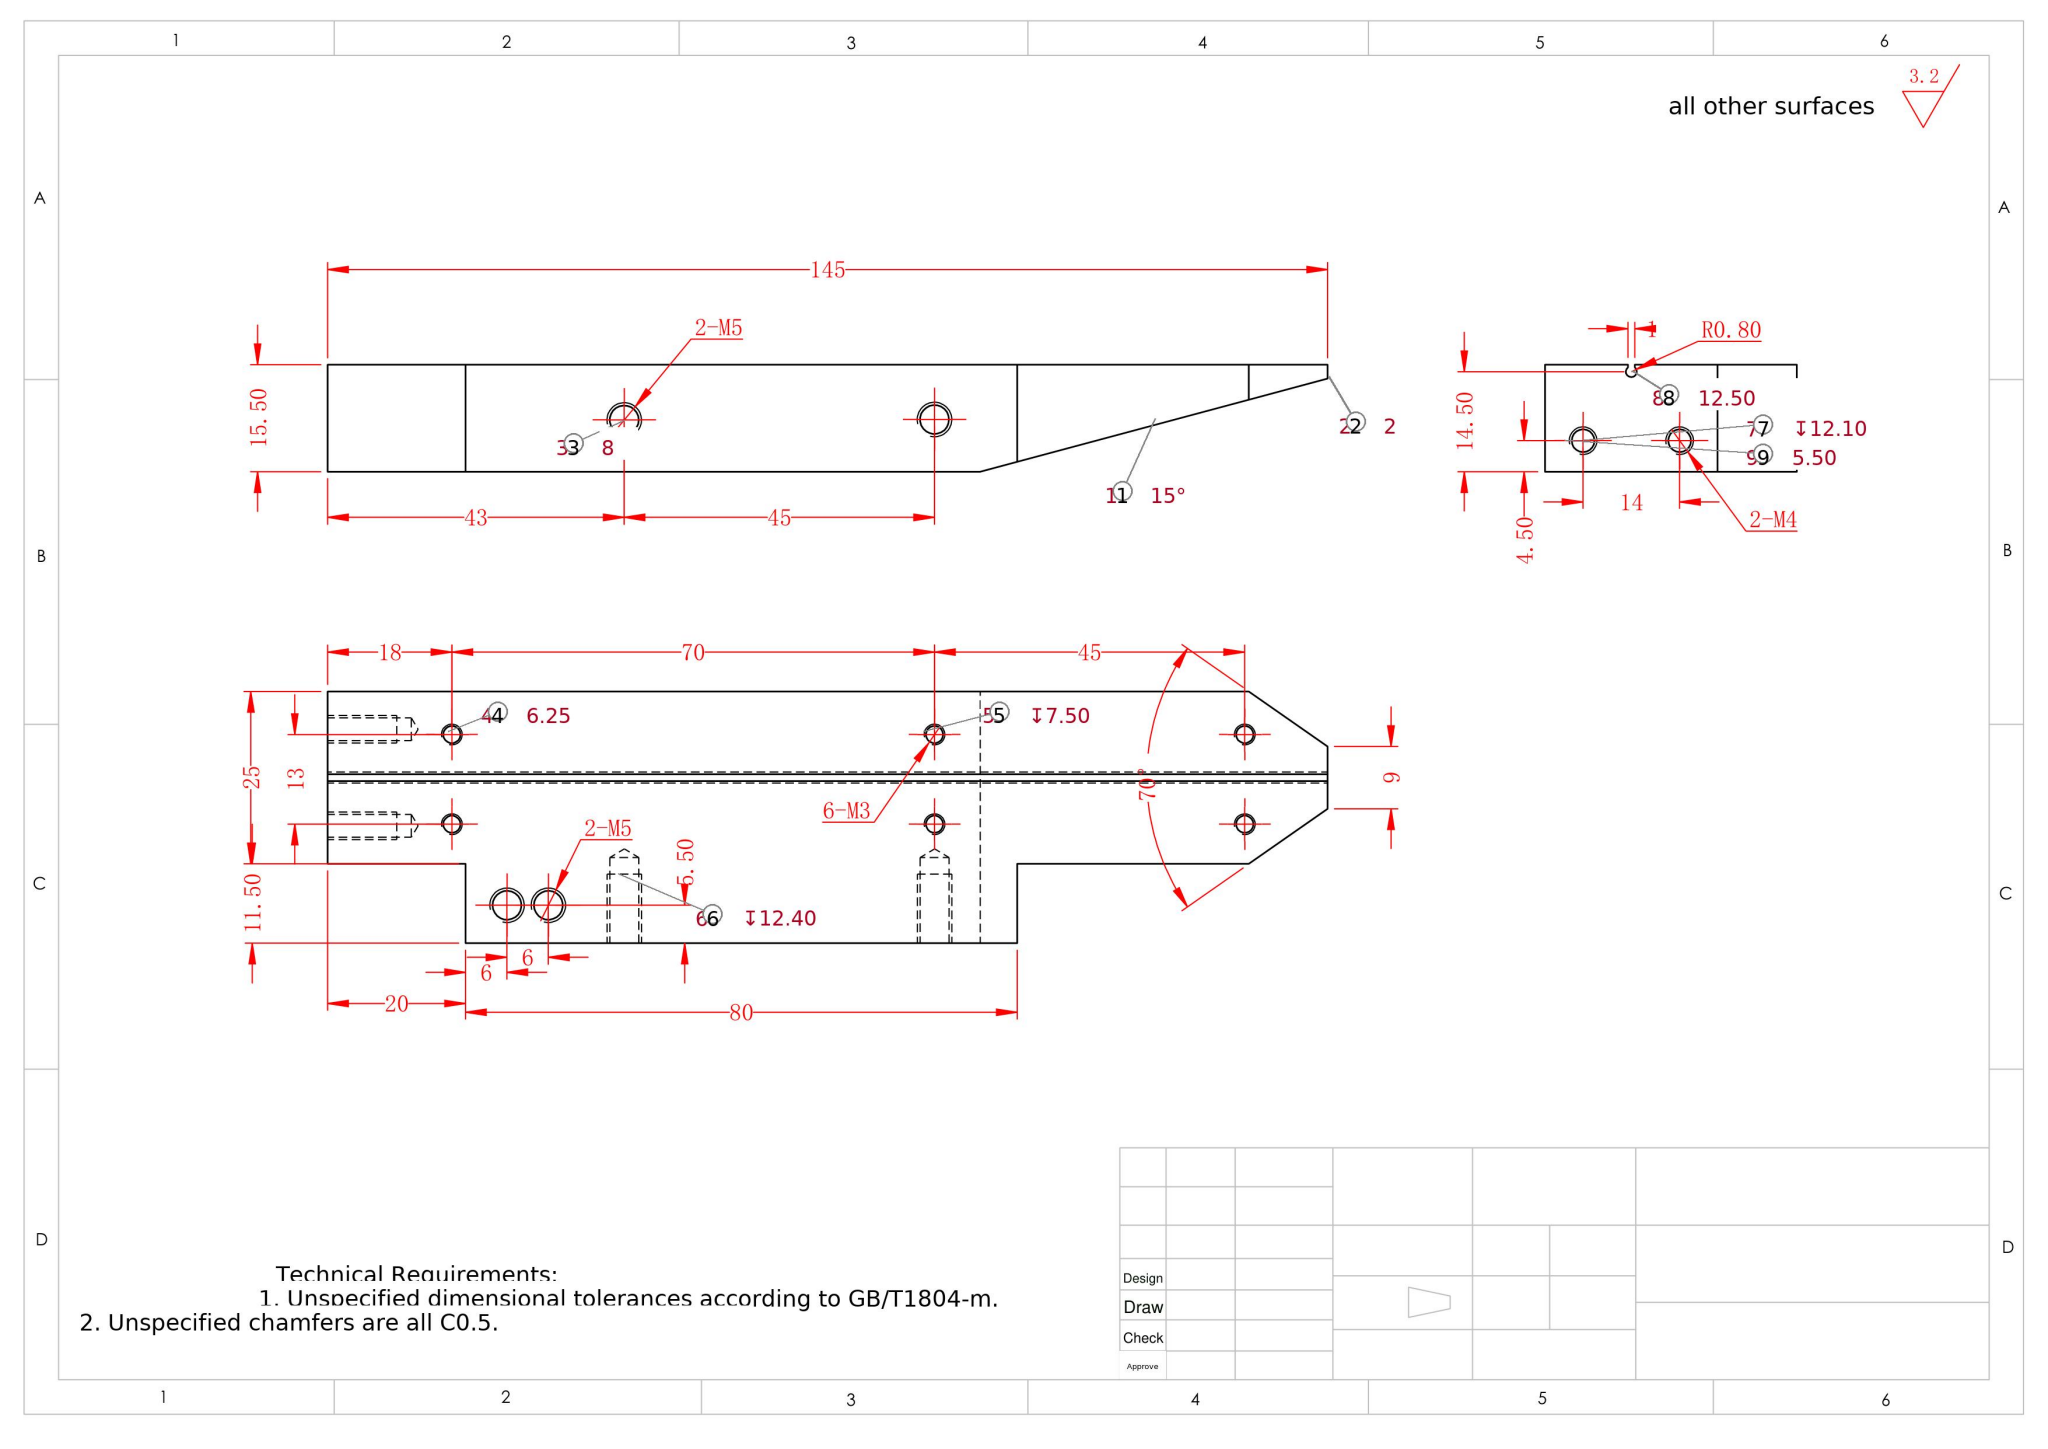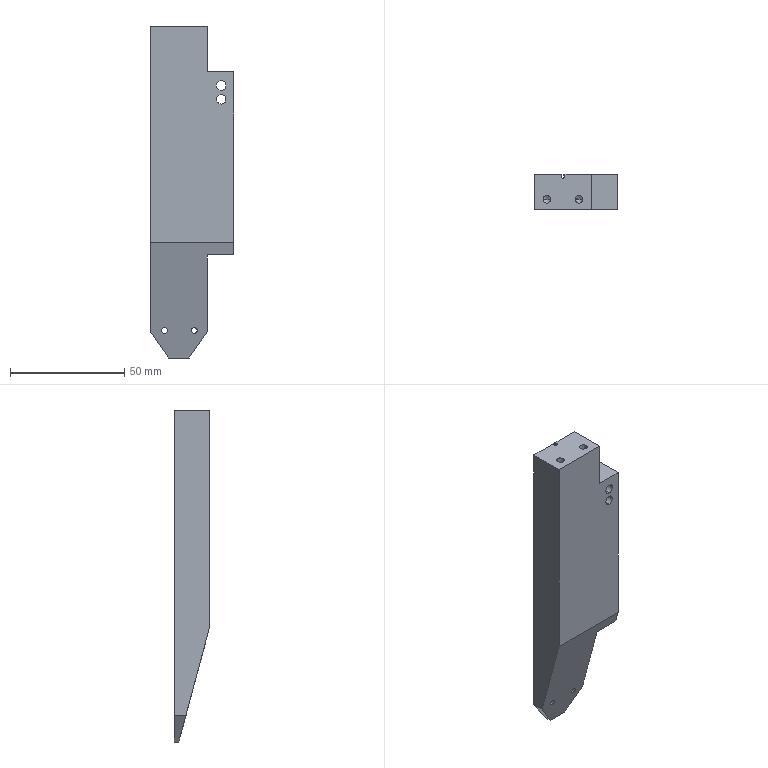Part | SolidWorks | mm | 1 solid | 59 faces | box 36.5 x 15.5 x 145 mm | volume 60095 mm3 | cylinder 27 | cone 16 | plane 16 | commonest cylinder face diameters 2.5 x12 4.2 x8 3.3 x4 1.6 x3
build123d program:
from build123d import *

# Parameters (mm, degrees)
BOSS_EXTRUDE1_DEPTH   = 145
CHAMFER1_SIZE         = 8
CHAMFER1_SIZE2        = 11.425
CUT_EXTRUDE1_REACH    = 150.461
M3_TAPPED_HOLE1_D     = 2.5
M3_TAPPED_HOLE1_DEPTH = 7.5
M3_TAPPED_HOLE1_TIP   = 0.7511
SKETCH15_W            = 80
SKETCH15_H            = 15.5
BOSS_EXTRUDE2_DEPTH   = 11.5
M4_TAPPED_HOLE5_D     = 3.3
M4_TAPPED_HOLE5_DEPTH = 12.1
M4_TAPPED_HOLE5_TIP   = 0.9914
M5_TAPPED_HOLE2_D     = 4.2
M5_TAPPED_HOLE2_DEPTH = 12.4
M5_TAPPED_HOLE2_TIP   = 1.262
M5_TAPPED_HOLE1_D     = 4.2
CUT_EXTRUDE2_DEPTH    = 149.461


with BuildPart() as part:
    # Sketch1 → Boss-Extrude1 (new body)
    with BuildSketch(Plane.XY):
        with BuildLine():
            Line((-29.862, 19.763), (-29.862, 4.263))
            Line((-29.862, 4.263), (-4.862, 4.263))
            Line((-4.862, 4.263), (-4.862, 19.763))
            Line((-4.862, 19.763), (-16.862, 19.763))
            Line((-16.862, 19.763), (-16.862, 19.388))
            ThreePointArc((-16.862, 19.388), (-17.362, 17.963), (-17.862, 19.388))
            Line((-17.862, 19.388), (-17.862, 19.763))
            Line((-17.862, 19.763), (-29.862, 19.763))
        make_face()
    extrude(amount=BOSS_EXTRUDE1_DEPTH)

    # Chamfer1
    chamfer1_edges = [part.edges().sort_by_distance(p)[0] for p in [
        (-29.862, 12.013, 0),
        (-4.862, 12.013, 0),
    ]]
    chamfer1_side = [part.faces().sort_by_distance(p)[0] for p in [
        (-17.362, 11.973, 0),
    ]]
    chamfer(chamfer1_edges, length=CHAMFER1_SIZE, length2=CHAMFER1_SIZE2, reference=chamfer1_side[0])

    # Sketch5 → Cut-Extrude1 (cut, up to next)
    with BuildSketch(Plane.ZY.offset(29.862), mode=Mode.PRIVATE) as cut_extrude1_sk1:
        Polygon((0, 17.763), (55, 3.026), (55, -2.385), (-1.143, -3.33), align=None)
    cut_extrude1_tool1 = extrude(cut_extrude1_sk1.sketch, amount=-CUT_EXTRUDE1_REACH, mode=Mode.PRIVATE) & part.part
    add(cut_extrude1_tool1.solids().sort_by_distance((-29.862, 4.442, 21.714))[0], mode=Mode.SUBTRACT)

    # M3 Tapped Hole1
    with Locations(Plane(origin=(0, 19.763, 0), x_dir=(1, 0, 0), z_dir=(0, 1, 0))):
        with Locations((-10.612, -12), (-23.612, -12), (-10.612, -57), (-23.612, -57), (-23.612, -127), (-10.612, -127)):
            Hole(M3_TAPPED_HOLE1_D / 2, depth=M3_TAPPED_HOLE1_DEPTH)
            with Locations((0, 0, -(M3_TAPPED_HOLE1_DEPTH + M3_TAPPED_HOLE1_TIP / 2))):  # 118° drill point
                Cone(0, M3_TAPPED_HOLE1_D / 2, M3_TAPPED_HOLE1_TIP, mode=Mode.SUBTRACT)

    # Sketch15 → Boss-Extrude2 (add)
    with BuildSketch(Plane(origin=(-4.862, 0, 0), x_dir=(0, 0, -1), z_dir=(1, 0, 0))):
        with Locations((-85, 12.013)):
            Rectangle(SKETCH15_W, SKETCH15_H)
    extrude(amount=BOSS_EXTRUDE2_DEPTH)

    # M4 Tapped Hole5
    with Locations(Plane.XY.offset(145)):
        with Locations((-24.362, 8.763), (-10.362, 8.763)):
            Hole(M4_TAPPED_HOLE5_D / 2, depth=M4_TAPPED_HOLE5_DEPTH)
            with Locations((0, 0, -(M4_TAPPED_HOLE5_DEPTH + M4_TAPPED_HOLE5_TIP / 2))):  # 118° drill point
                Cone(0, M4_TAPPED_HOLE5_D / 2, M4_TAPPED_HOLE5_TIP, mode=Mode.SUBTRACT)

    # M5 Tapped Hole2
    with Locations(Plane(origin=(6.638, 0, 0), x_dir=(0, 0, -1), z_dir=(1, 0, 0))):
        with Locations((-102, 11.763), (-57, 11.829)):
            Hole(M5_TAPPED_HOLE2_D / 2, depth=M5_TAPPED_HOLE2_DEPTH)
            with Locations((0, 0, -(M5_TAPPED_HOLE2_DEPTH + M5_TAPPED_HOLE2_TIP / 2))):  # 118° drill point
                Cone(0, M5_TAPPED_HOLE2_D / 2, M5_TAPPED_HOLE2_TIP, mode=Mode.SUBTRACT)

    # M5 Tapped Hole1 (through all)
    with Locations(Plane(origin=(0, 19.763, 0), x_dir=(1, 0, 0), z_dir=(0, 1, 0))):
        with Locations((1.138, -119), (1.138, -113)):
            Hole(M5_TAPPED_HOLE1_D / 2)

    # Sketch30 → Cut-Extrude2 (cut, through all)
    with BuildSketch(Plane.ZY.offset(4.862)):
        Polygon((45, 5.706), (50.383, 4.263), (45, 4.263), align=None)
    extrude(amount=-CUT_EXTRUDE2_DEPTH, mode=Mode.SUBTRACT)


solid = part.part